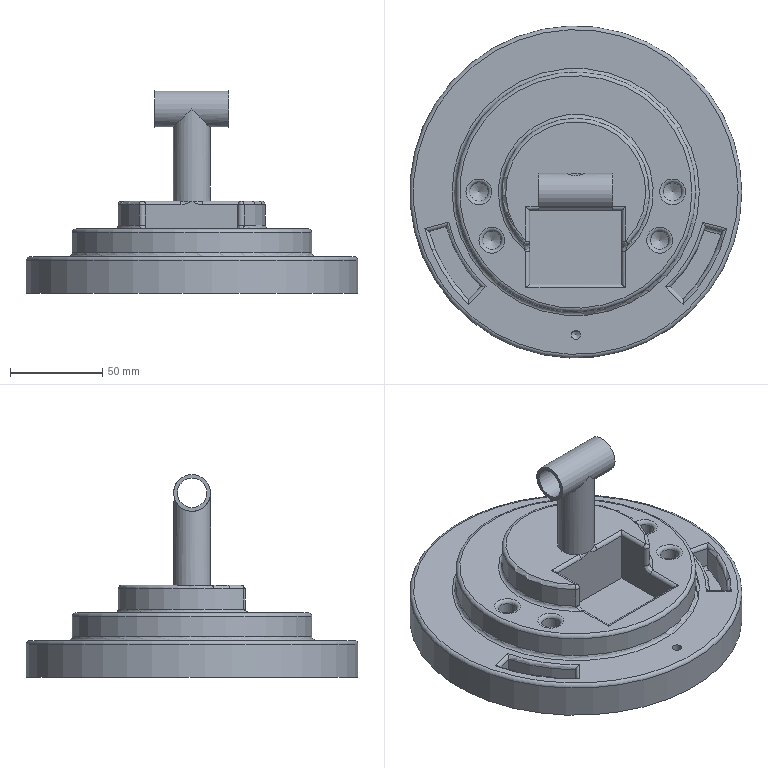Component | NX | BASE_PLATE | 1 solid | 80 faces | volume 726098 mm3 | cylinder 33 | plane 20 | torus 13 | spline 7 | cone 5 | sphere 2 | commonest cylinder face diameters 4 x14 10 x5 8.5 x2 5 x2 20 x2 164.455 x2 145.456 x2 180 x1